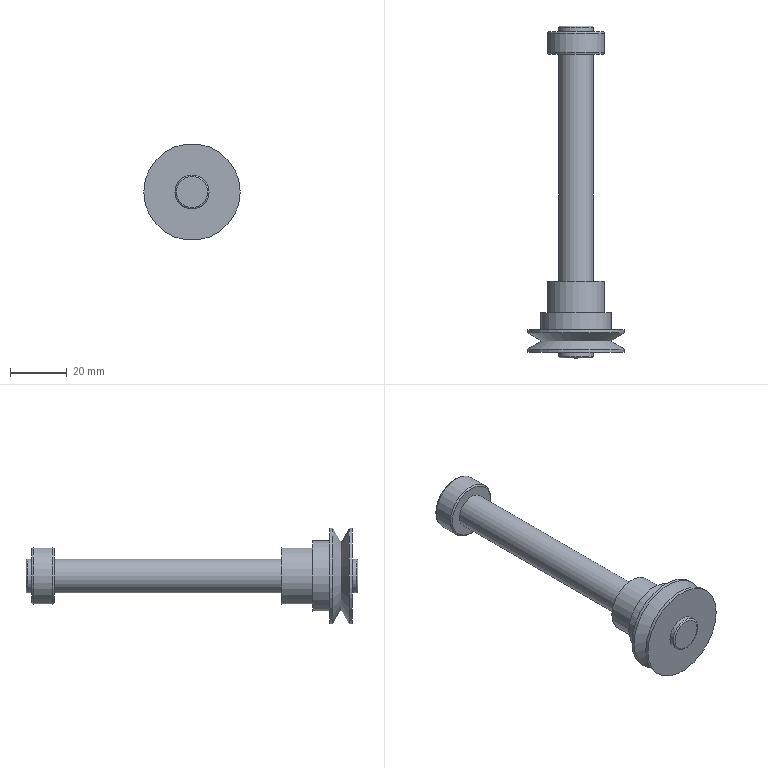Component | NX | MOTOR_SHAFT | 1 solid | 22 faces | volume 24277 mm3 | plane 8 | cylinder 8 | torus 4 | cone 2 | commonest cylinder face diameters 12 x3 20 x2 34 x2 25 x1